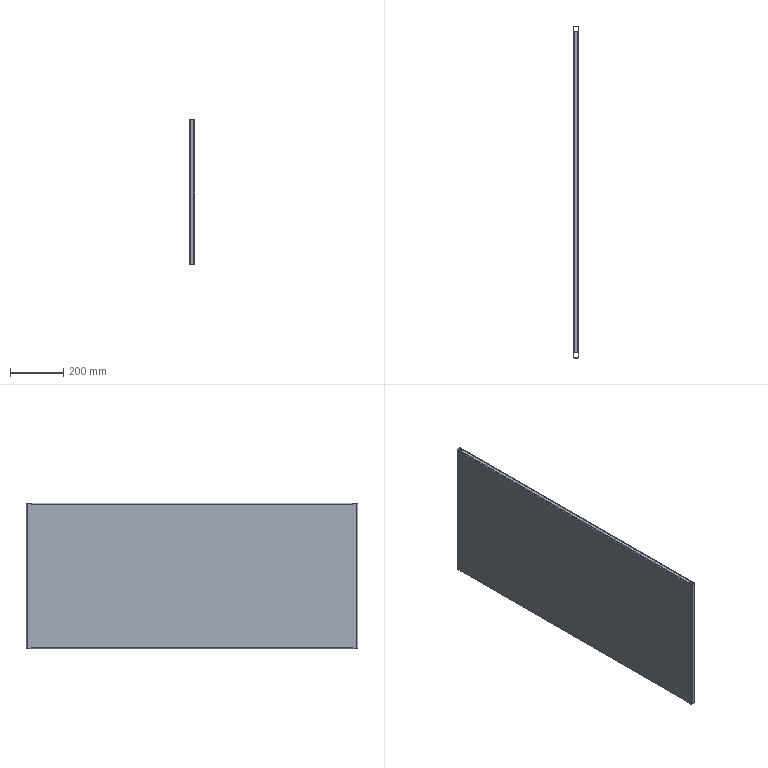Component | SolidWorks | RearDoor-2 | 1 solid | 86 faces | volume 1574835 mm3 | plane 70 | cylinder 16 | commonest cylinder face diameters 8 x8 4 x8